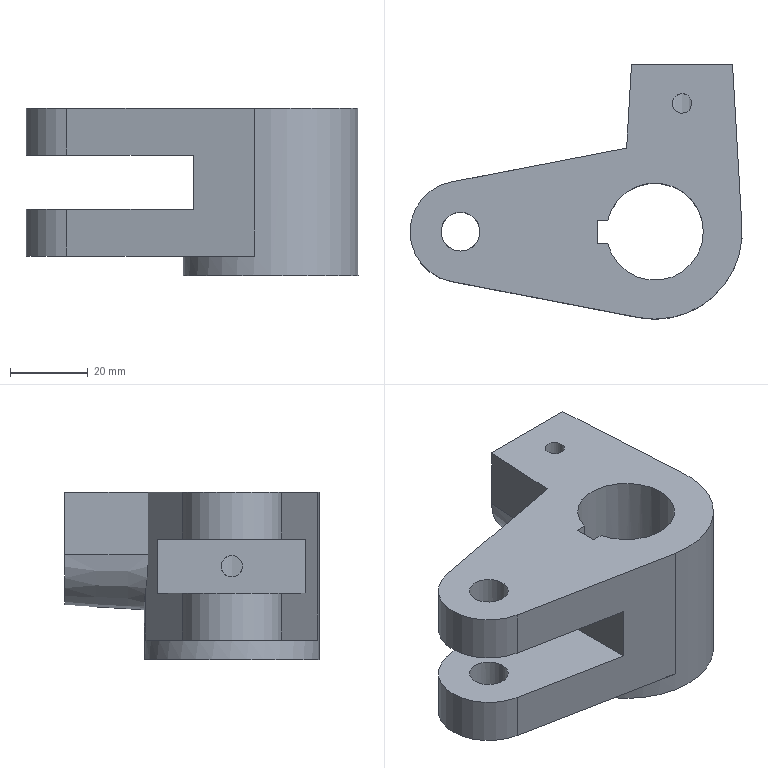Component | NX | HANDLE_BASE | 1 solid | 27 faces | volume 88532 mm3 | plane 15 | cylinder 10 | cone 1 | spline 1 | commonest cylinder face diameters 26 x2 10 x2 14 x1 25 x1 45 x1 5 x1 9 x1 5.5 x1